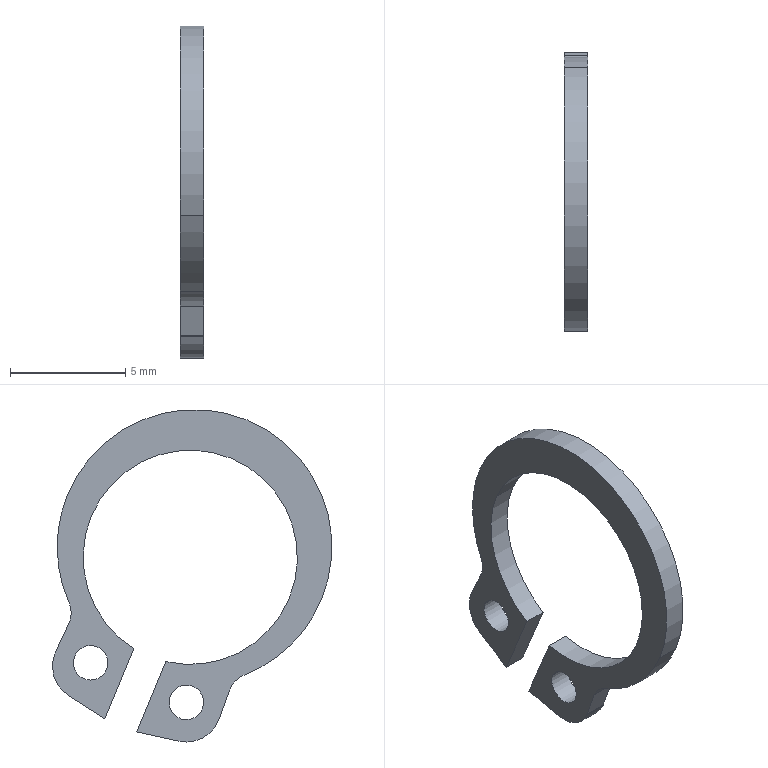Component | NX | CIRCLIP_SHAFT_A10 | 1 solid | 24 faces | volume 55 mm3 | cylinder 16 | plane 8 | commonest cylinder face diameters 1.5 x4 2.2 x3 9.3 x3 3 x3 11.925 x3